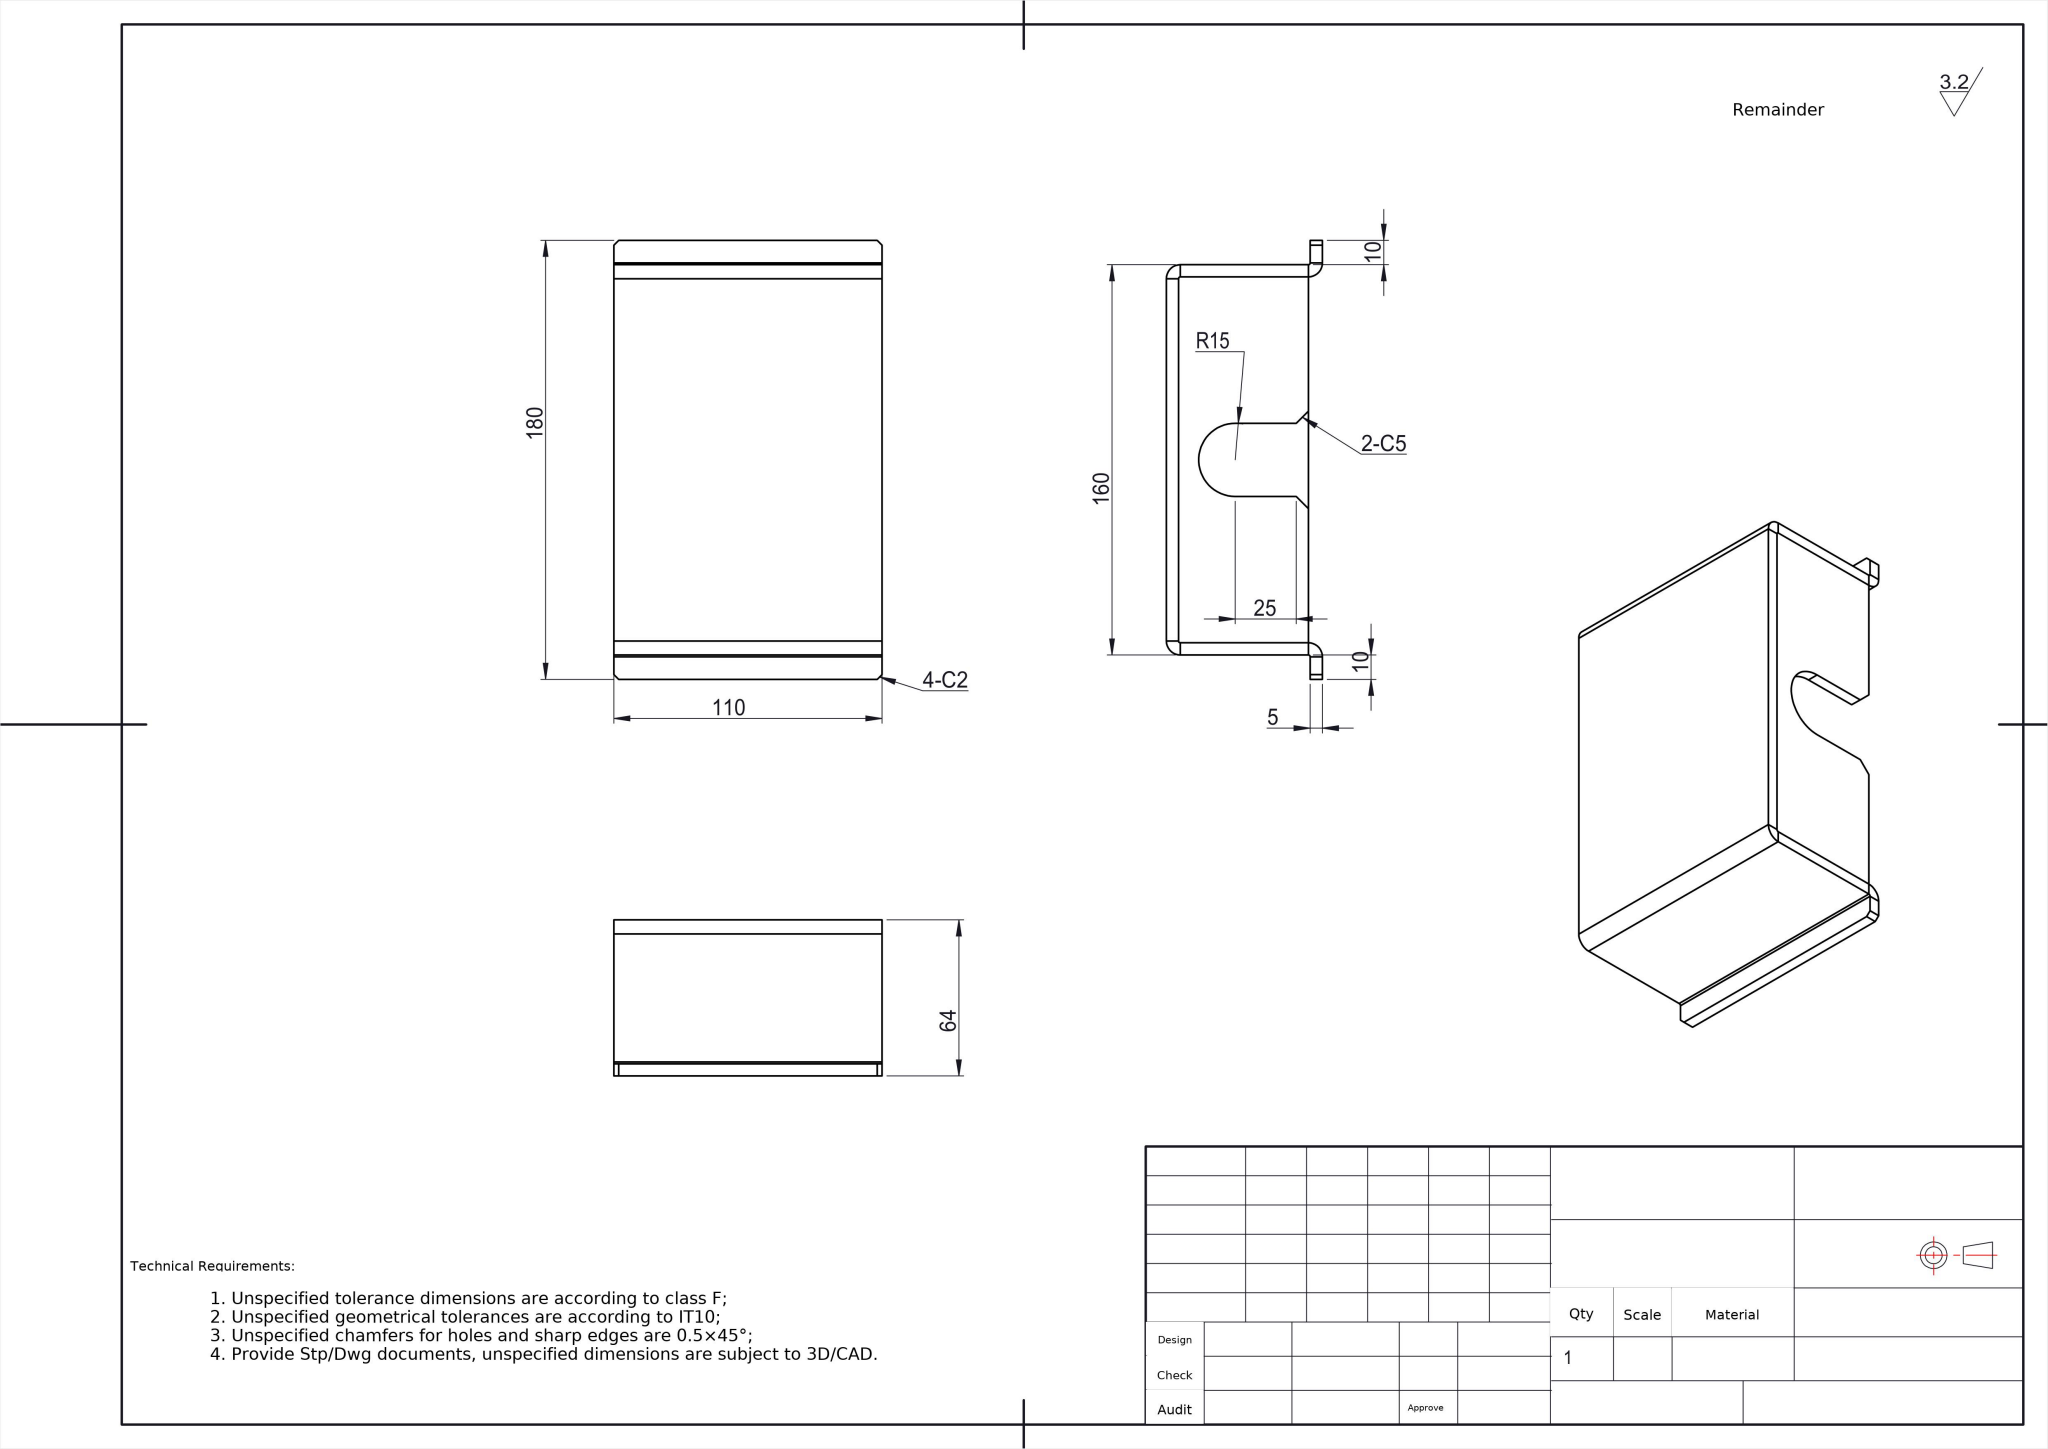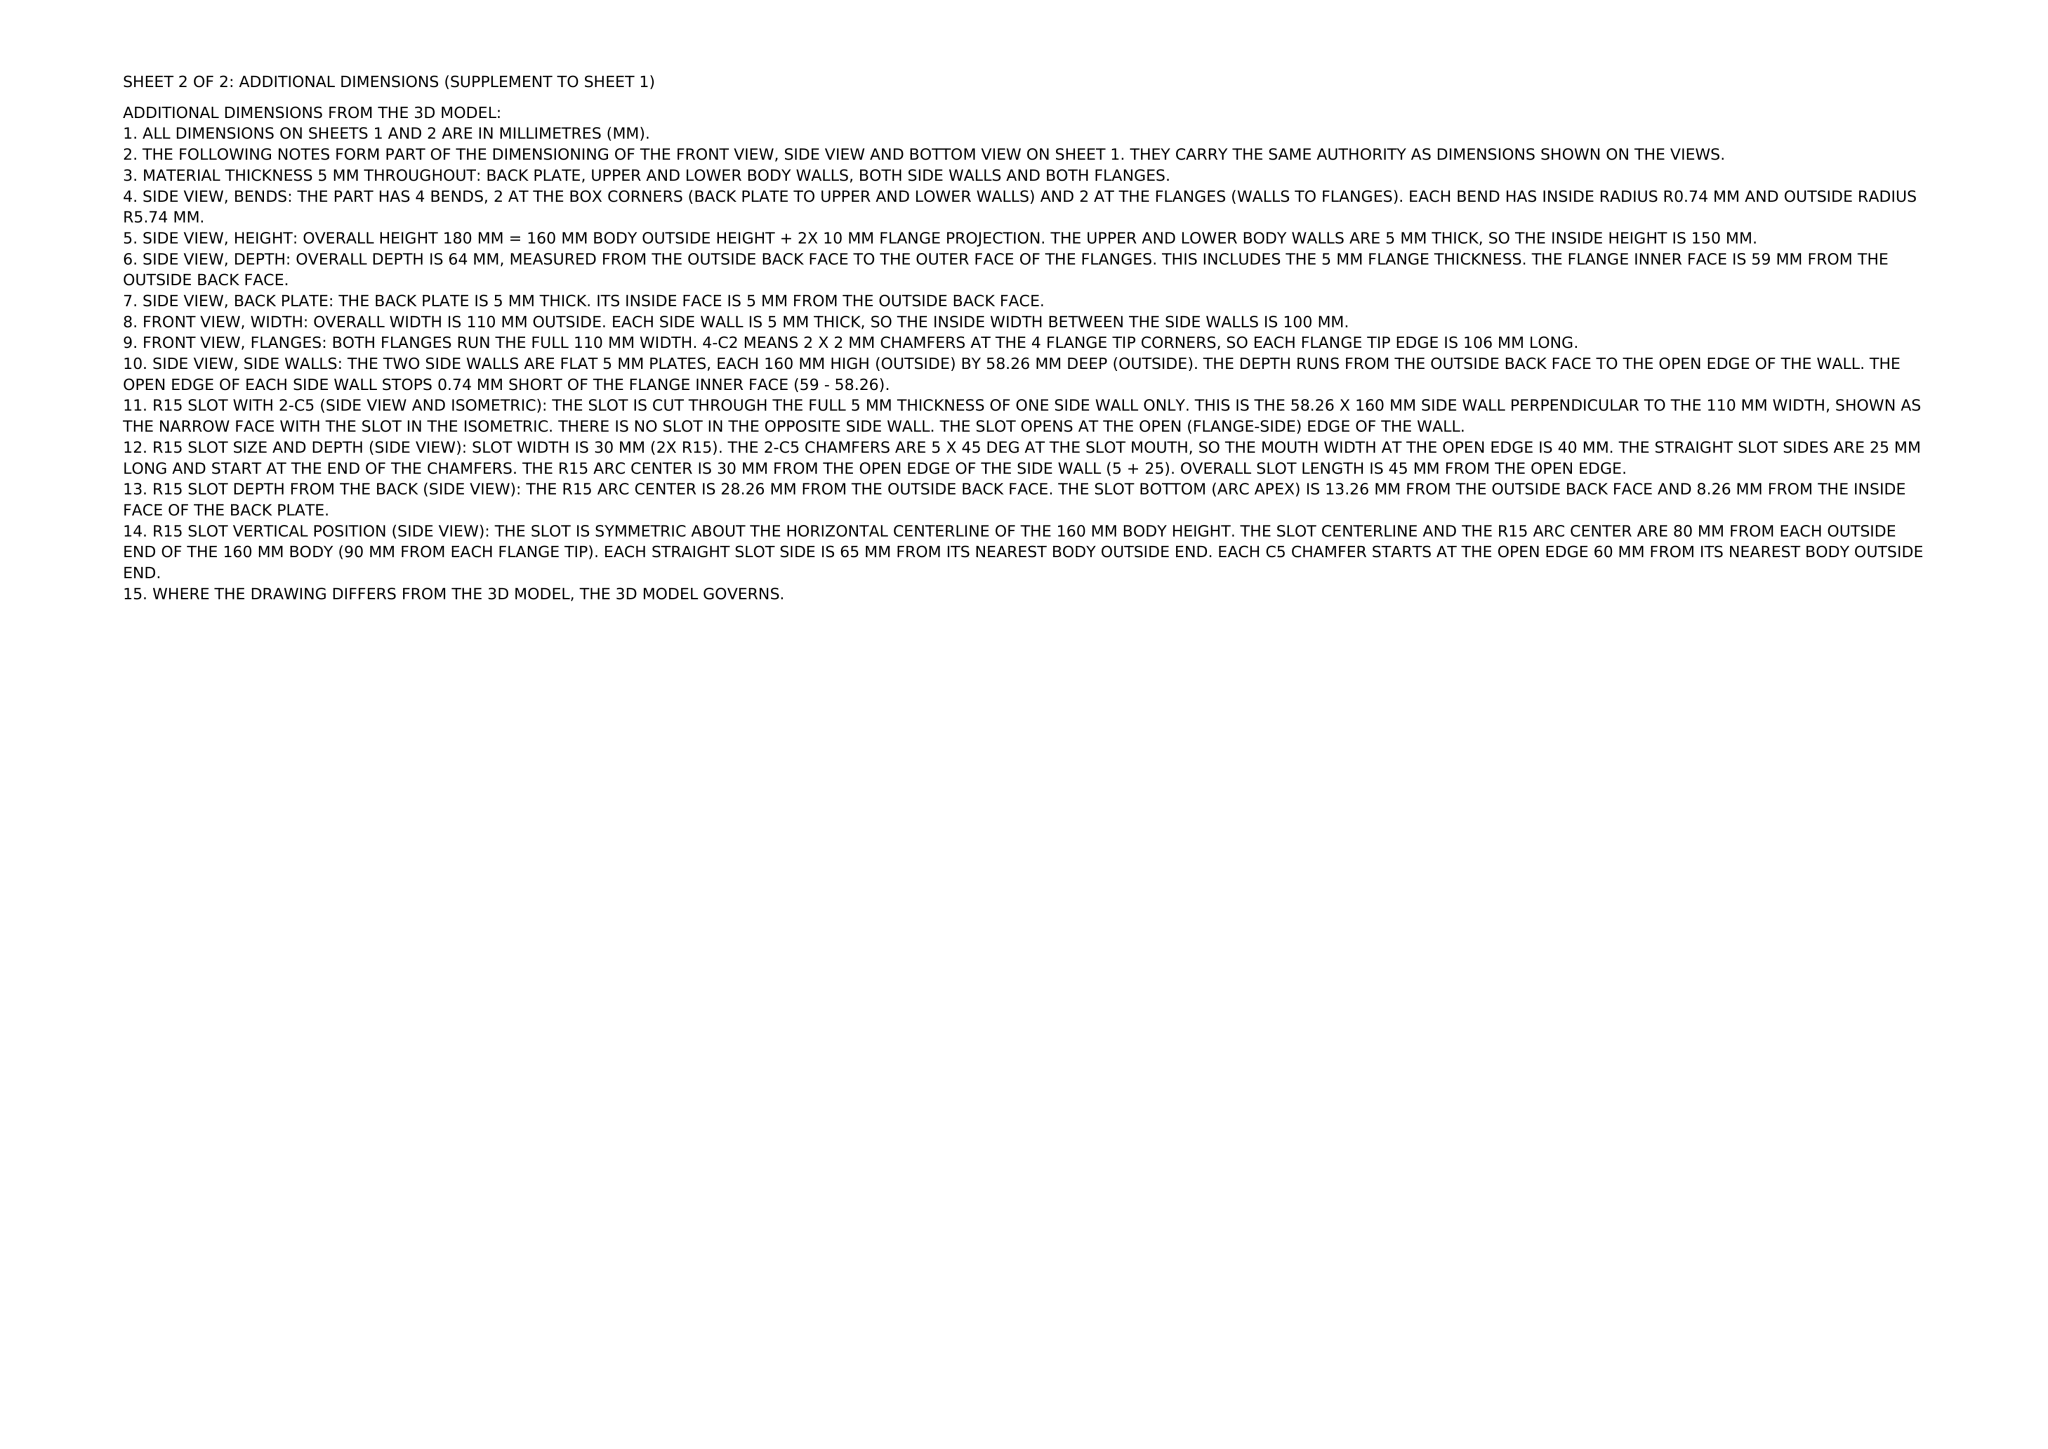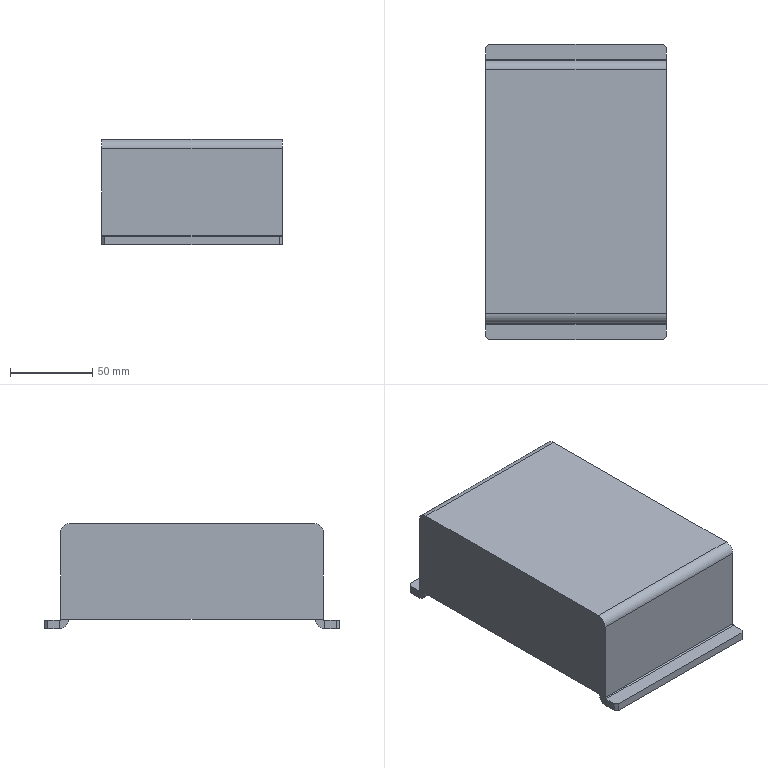Part | NX | mm | 1 solid | 44 faces | box 110 x 180 x 64 mm | volume 234304 mm3 | plane 35 | cylinder 9 | commonest cylinder face diameters 1.473 x4 11.473 x4 30 x1